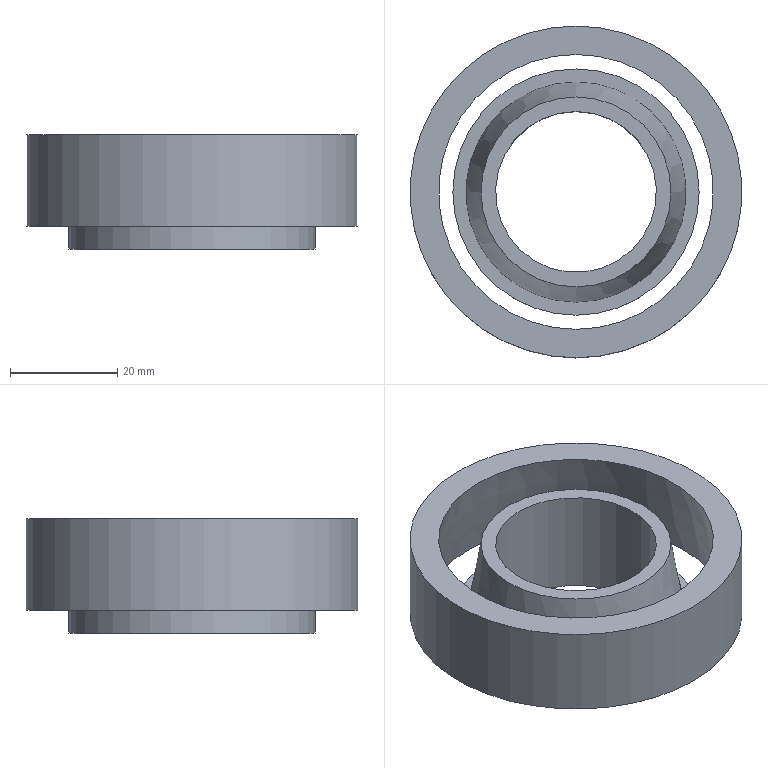Component | NX | GUNZIZGOUCHOU2 | 2 solids | 10 faces | box 61.88 x 61.88 x 21.26 mm | volume 22800 mm3 | plane 5 | cylinder 3 | cone 2 | commonest cylinder face diameters 61.88 x1 30 x1 45.92 x1
STEP:
#1=CARTESIAN_POINT('',(0.,0.,0.));
#2=DIRECTION('',(0.,0.,1.));
#3=DIRECTION('',(1.,0.,0.));
#4=AXIS2_PLACEMENT_3D('',#1,#2,#3);
#5=CARTESIAN_POINT('',(0.,28.646,365.26));
#6=VERTEX_POINT('',#5);
#7=CARTESIAN_POINT('',(0.,0.,365.26));
#8=DIRECTION('',(0.,0.,-1.));
#9=DIRECTION('',(0.,1.,0.));
#10=AXIS2_PLACEMENT_3D('',#7,#8,#9);
#11=CIRCLE('',#10,28.646);
#12=CARTESIAN_POINT('',(0.,0.,366.664));
#13=DIRECTION('',(0.,0.,-1.));
#14=DIRECTION('',(0.,1.,0.));
#15=AXIS2_PLACEMENT_3D('',#12,#13,#14);
#16=CONICAL_SURFACE('',#15,28.396,0.1764);
#17=CARTESIAN_POINT('',(0.,1.404));
#18=DIRECTION('',(1.,0.));
#19=VECTOR('',#18,1.);
#20=LINE('',#17,#19);
#21=(GEOMETRIC_REPRESENTATION_CONTEXT(2)PARAMETRIC_REPRESENTATION_CONTEXT()REPRESENTATION_CONTEXT('',''));
#22=DEFINITIONAL_REPRESENTATION('',(#20),#21);
#23=PCURVE('',#16,#22);
#24=CARTESIAN_POINT('',(28.646,0.,365.26));
#25=DIRECTION('',(0.,0.,-1.));
#26=DIRECTION('',(0.,1.,0.));
#27=AXIS2_PLACEMENT_3D('',#24,#25,#26);
#28=PLANE('',#27);
#29=CARTESIAN_POINT('',(0.,-28.646));
#30=DIRECTION('',(1.,0.));
#31=AXIS2_PLACEMENT_2D('',#29,#30);
#32=CIRCLE('',#31,28.646);
#33=(GEOMETRIC_REPRESENTATION_CONTEXT(2)PARAMETRIC_REPRESENTATION_CONTEXT()REPRESENTATION_CONTEXT('',''));
#34=DEFINITIONAL_REPRESENTATION('',(#32),#33);
#35=PCURVE('',#28,#34);
#36=SURFACE_CURVE('',#11,(#23,#35),.PCURVE_S1.);
#37=EDGE_CURVE('',#6,#6,#36,.T.);
#38=ORIENTED_EDGE('',*,*,#37,.F.);
#39=CARTESIAN_POINT('',(0.,25.616,382.26));
#40=VERTEX_POINT('',#39);
#41=CARTESIAN_POINT('',(-0.,25.616,382.26));
#42=CARTESIAN_POINT('',(-0.,28.646,365.26));
#43=B_SPLINE_CURVE_WITH_KNOTS('',1,(#41,#42),.UNSPECIFIED.,.F.,.F.,(2,2),(-15.842,1.426),.PIECEWISE_BEZIER_KNOTS.);
#44=CARTESIAN_POINT('',(0.,0.));
#45=DIRECTION('',(0.,1.));
#46=VECTOR('',#45,1.);
#47=LINE('',#44,#46);
#48=(GEOMETRIC_REPRESENTATION_CONTEXT(2)PARAMETRIC_REPRESENTATION_CONTEXT()REPRESENTATION_CONTEXT('',''));
#49=DEFINITIONAL_REPRESENTATION('',(#47),#48);
#50=PCURVE('',#16,#49);
#51=CARTESIAN_POINT('',(6.283,0.));
#52=DIRECTION('',(0.,1.));
#53=VECTOR('',#52,1.);
#54=LINE('',#51,#53);
#55=(GEOMETRIC_REPRESENTATION_CONTEXT(2)PARAMETRIC_REPRESENTATION_CONTEXT()REPRESENTATION_CONTEXT('',''));
#56=DEFINITIONAL_REPRESENTATION('',(#54),#55);
#57=PCURVE('',#16,#56);
#58=SEAM_CURVE('',#43,(#50,#57),.PCURVE_S1.);
#59=EDGE_CURVE('',#40,#6,#58,.T.);
#60=ORIENTED_EDGE('',*,*,#59,.F.);
#61=CARTESIAN_POINT('',(0.,0.,382.26));
#62=DIRECTION('',(0.,0.,-1.));
#63=DIRECTION('',(0.,1.,0.));
#64=AXIS2_PLACEMENT_3D('',#61,#62,#63);
#65=CIRCLE('',#64,25.616);
#66=CARTESIAN_POINT('',(0.,-15.596));
#67=DIRECTION('',(1.,0.));
#68=VECTOR('',#67,1.);
#69=LINE('',#66,#68);
#70=(GEOMETRIC_REPRESENTATION_CONTEXT(2)PARAMETRIC_REPRESENTATION_CONTEXT()REPRESENTATION_CONTEXT('',''));
#71=DEFINITIONAL_REPRESENTATION('',(#69),#70);
#72=PCURVE('',#16,#71);
#73=CARTESIAN_POINT('',(27.255,0.,382.26));
#74=DIRECTION('',(0.,0.,1.));
#75=DIRECTION('',(0.,-1.,0.));
#76=AXIS2_PLACEMENT_3D('',#73,#74,#75);
#77=PLANE('',#76);
#78=CARTESIAN_POINT('',(-25.616,-27.255));
#79=CARTESIAN_POINT('',(-25.616,17.113));
#80=CARTESIAN_POINT('',(12.808,-5.071));
#81=CARTESIAN_POINT('',(51.232,-27.255));
#82=CARTESIAN_POINT('',(12.808,-49.439));
#83=CARTESIAN_POINT('',(-25.616,-71.623));
#84=CARTESIAN_POINT('',(-25.616,-27.255));
#85=(BOUNDED_CURVE()B_SPLINE_CURVE(2,(#78,#79,#80,#81,#82,#83,#84),.UNSPECIFIED.,.T.,.F.)B_SPLINE_CURVE_WITH_KNOTS((1,2,2,2,2,1),(-2.094,0.,2.094,4.189,6.283,8.378),.UNSPECIFIED.)CURVE()GEOMETRIC_REPRESENTATION_ITEM()RATIONAL_B_SPLINE_CURVE((1.,0.5,1.,0.5,1.,0.5,1.))REPRESENTATION_ITEM(''));
#86=(GEOMETRIC_REPRESENTATION_CONTEXT(2)PARAMETRIC_REPRESENTATION_CONTEXT()REPRESENTATION_CONTEXT('',''));
#87=DEFINITIONAL_REPRESENTATION('',(#85),#86);
#88=PCURVE('',#77,#87);
#89=SURFACE_CURVE('',#65,(#72,#88),.PCURVE_S1.);
#90=EDGE_CURVE('',#40,#40,#89,.T.);
#91=ORIENTED_EDGE('',*,*,#90,.T.);
#92=ORIENTED_EDGE('',*,*,#59,.T.);
#93=EDGE_LOOP('',(#38,#60,#91,#92));
#94=FACE_BOUND('',#93,.F.);
#95=ADVANCED_FACE('',(#94),#16,.F.);
#96=CARTESIAN_POINT('',(0.,30.94,365.26));
#97=VERTEX_POINT('',#96);
#98=CARTESIAN_POINT('',(0.,0.,365.26));
#99=DIRECTION('',(0.,0.,-1.));
#100=DIRECTION('',(0.,1.,0.));
#101=AXIS2_PLACEMENT_3D('',#98,#99,#100);
#102=CIRCLE('',#101,30.94);
#103=CARTESIAN_POINT('',(0.,-28.646));
#104=DIRECTION('',(1.,0.));
#105=AXIS2_PLACEMENT_2D('',#103,#104);
#106=CIRCLE('',#105,30.94);
#107=(GEOMETRIC_REPRESENTATION_CONTEXT(2)PARAMETRIC_REPRESENTATION_CONTEXT()REPRESENTATION_CONTEXT('',''));
#108=DEFINITIONAL_REPRESENTATION('',(#106),#107);
#109=PCURVE('',#28,#108);
#110=CARTESIAN_POINT('',(0.,0.,361.));
#111=DIRECTION('',(0.,0.,-1.));
#112=DIRECTION('',(0.,1.,0.));
#113=AXIS2_PLACEMENT_3D('',#110,#111,#112);
#114=CYLINDRICAL_SURFACE('',#113,30.94);
#115=CARTESIAN_POINT('',(0.,-4.26));
#116=DIRECTION('',(1.,0.));
#117=VECTOR('',#116,1.);
#118=LINE('',#115,#117);
#119=(GEOMETRIC_REPRESENTATION_CONTEXT(2)PARAMETRIC_REPRESENTATION_CONTEXT()REPRESENTATION_CONTEXT('',''));
#120=DEFINITIONAL_REPRESENTATION('',(#118),#119);
#121=PCURVE('',#114,#120);
#122=SURFACE_CURVE('',#102,(#109,#121),.PCURVE_S1.);
#123=EDGE_CURVE('',#97,#97,#122,.T.);
#124=ORIENTED_EDGE('',*,*,#123,.T.);
#125=EDGE_LOOP('',(#124));
#126=FACE_BOUND('',#125,.T.);
#127=ORIENTED_EDGE('',*,*,#37,.F.);
#128=EDGE_LOOP('',(#127));
#129=FACE_BOUND('',#128,.T.);
#130=ADVANCED_FACE('',(#126,#129),#28,.T.);
#131=CARTESIAN_POINT('',(0.,30.94,382.26));
#132=VERTEX_POINT('',#131);
#133=CARTESIAN_POINT('',(0.,0.,382.26));
#134=DIRECTION('',(0.,0.,-1.));
#135=DIRECTION('',(0.,1.,0.));
#136=AXIS2_PLACEMENT_3D('',#133,#134,#135);
#137=CIRCLE('',#136,30.94);
#138=CARTESIAN_POINT('',(0.,-21.26));
#139=DIRECTION('',(1.,0.));
#140=VECTOR('',#139,1.);
#141=LINE('',#138,#140);
#142=(GEOMETRIC_REPRESENTATION_CONTEXT(2)PARAMETRIC_REPRESENTATION_CONTEXT()REPRESENTATION_CONTEXT('',''));
#143=DEFINITIONAL_REPRESENTATION('',(#141),#142);
#144=PCURVE('',#114,#143);
#145=CARTESIAN_POINT('',(-30.94,-27.255));
#146=CARTESIAN_POINT('',(-30.94,26.334));
#147=CARTESIAN_POINT('',(15.47,-0.4604));
#148=CARTESIAN_POINT('',(61.88,-27.255));
#149=CARTESIAN_POINT('',(15.47,-54.05));
#150=CARTESIAN_POINT('',(-30.94,-80.845));
#151=CARTESIAN_POINT('',(-30.94,-27.255));
#152=(BOUNDED_CURVE()B_SPLINE_CURVE(2,(#145,#146,#147,#148,#149,#150,#151),.UNSPECIFIED.,.T.,.F.)B_SPLINE_CURVE_WITH_KNOTS((1,2,2,2,2,1),(-2.094,0.,2.094,4.189,6.283,8.378),.UNSPECIFIED.)CURVE()GEOMETRIC_REPRESENTATION_ITEM()RATIONAL_B_SPLINE_CURVE((1.,0.5,1.,0.5,1.,0.5,1.))REPRESENTATION_ITEM(''));
#153=(GEOMETRIC_REPRESENTATION_CONTEXT(2)PARAMETRIC_REPRESENTATION_CONTEXT()REPRESENTATION_CONTEXT('',''));
#154=DEFINITIONAL_REPRESENTATION('',(#152),#153);
#155=PCURVE('',#77,#154);
#156=SURFACE_CURVE('',#137,(#144,#155),.PCURVE_S1.);
#157=EDGE_CURVE('',#132,#132,#156,.T.);
#158=ORIENTED_EDGE('',*,*,#157,.T.);
#159=CARTESIAN_POINT('',(0.,30.94,382.26));
#160=CARTESIAN_POINT('',(0.,30.94,365.26));
#161=B_SPLINE_CURVE_WITH_KNOTS('',1,(#159,#160),.UNSPECIFIED.,.F.,.F.,(2,2),(-21.26,-4.26),.PIECEWISE_BEZIER_KNOTS.);
#162=CARTESIAN_POINT('',(6.283,0.));
#163=DIRECTION('',(0.,1.));
#164=VECTOR('',#163,1.);
#165=LINE('',#162,#164);
#166=(GEOMETRIC_REPRESENTATION_CONTEXT(2)PARAMETRIC_REPRESENTATION_CONTEXT()REPRESENTATION_CONTEXT('',''));
#167=DEFINITIONAL_REPRESENTATION('',(#165),#166);
#168=PCURVE('',#114,#167);
#169=CARTESIAN_POINT('',(0.,0.));
#170=DIRECTION('',(0.,1.));
#171=VECTOR('',#170,1.);
#172=LINE('',#169,#171);
#173=(GEOMETRIC_REPRESENTATION_CONTEXT(2)PARAMETRIC_REPRESENTATION_CONTEXT()REPRESENTATION_CONTEXT('',''));
#174=DEFINITIONAL_REPRESENTATION('',(#172),#173);
#175=PCURVE('',#114,#174);
#176=SEAM_CURVE('',#161,(#168,#175),.PCURVE_S1.);
#177=EDGE_CURVE('',#132,#97,#176,.T.);
#178=ORIENTED_EDGE('',*,*,#177,.T.);
#179=ORIENTED_EDGE('',*,*,#123,.F.);
#180=ORIENTED_EDGE('',*,*,#177,.F.);
#181=EDGE_LOOP('',(#158,#178,#179,#180));
#182=FACE_BOUND('',#181,.T.);
#183=ADVANCED_FACE('',(#182),#114,.T.);
#184=ORIENTED_EDGE('',*,*,#90,.T.);
#185=EDGE_LOOP('',(#184));
#186=FACE_BOUND('',#185,.T.);
#187=ORIENTED_EDGE('',*,*,#157,.F.);
#188=EDGE_LOOP('',(#187));
#189=FACE_BOUND('',#188,.T.);
#190=ADVANCED_FACE('',(#186,#189),#77,.T.);
#191=CLOSED_SHELL('',(#95,#130,#183,#190));
#192=MANIFOLD_SOLID_BREP('',#191);
#193=(LENGTH_UNIT()NAMED_UNIT(*)SI_UNIT(.MILLI.,.METRE.));
#194=UNCERTAINTY_MEASURE_WITH_UNIT(LENGTH_MEASURE(0.00001),#193,'','');
#195=(NAMED_UNIT(*)PLANE_ANGLE_UNIT()SI_UNIT($,.RADIAN.));
#196=(NAMED_UNIT(*)SI_UNIT($,.STERADIAN.)SOLID_ANGLE_UNIT());
#197=(GEOMETRIC_REPRESENTATION_CONTEXT(3)GLOBAL_UNCERTAINTY_ASSIGNED_CONTEXT((#194))GLOBAL_UNIT_ASSIGNED_CONTEXT((#193,#195,#196))REPRESENTATION_CONTEXT('',''));
#198=ADVANCED_BREP_SHAPE_REPRESENTATION('',(#4,#192),#197);
#199=CARTESIAN_POINT('',(0.,0.,0.));
#200=DIRECTION('',(0.,0.,1.));
#201=DIRECTION('',(1.,0.,0.));
#202=AXIS2_PLACEMENT_3D('',#199,#200,#201);
#203=CARTESIAN_POINT('',(0.,0.,0.));
#204=DIRECTION('',(0.,0.,1.));
#205=DIRECTION('',(1.,0.,0.));
#206=AXIS2_PLACEMENT_3D('',#203,#204,#205);
#207=(LENGTH_UNIT()NAMED_UNIT(*)SI_UNIT(.MILLI.,.METRE.));
#208=UNCERTAINTY_MEASURE_WITH_UNIT(LENGTH_MEASURE(0.00001),#207,'','');
#209=(NAMED_UNIT(*)PLANE_ANGLE_UNIT()SI_UNIT($,.RADIAN.));
#210=(NAMED_UNIT(*)SI_UNIT($,.STERADIAN.)SOLID_ANGLE_UNIT());
#211=(GEOMETRIC_REPRESENTATION_CONTEXT(3)GLOBAL_UNCERTAINTY_ASSIGNED_CONTEXT((#208))GLOBAL_UNIT_ASSIGNED_CONTEXT((#207,#209,#210))REPRESENTATION_CONTEXT('',''));
#212=SHAPE_REPRESENTATION('',(#4,#202,#206),#211);
#213=ITEM_DEFINED_TRANSFORMATION('','',#4,#202);
#214=(REPRESENTATION_RELATIONSHIP('','',#198,#212)REPRESENTATION_RELATIONSHIP_WITH_TRANSFORMATION(#213)SHAPE_REPRESENTATION_RELATIONSHIP());
#215=CARTESIAN_POINT('',(0.,15.,381.02));
#216=VERTEX_POINT('',#215);
#217=CARTESIAN_POINT('',(0.,0.,381.02));
#218=DIRECTION('',(0.,0.,-1.));
#219=DIRECTION('',(0.,1.,0.));
#220=AXIS2_PLACEMENT_3D('',#217,#218,#219);
#221=CIRCLE('',#220,15.);
#222=CARTESIAN_POINT('',(17.711,0.,381.02));
#223=DIRECTION('',(0.,0.,1.));
#224=DIRECTION('',(0.,-1.,0.));
#225=AXIS2_PLACEMENT_3D('',#222,#223,#224);
#226=PLANE('',#225);
#227=CARTESIAN_POINT('',(-15.,-17.711));
#228=CARTESIAN_POINT('',(-15.,8.27));
#229=CARTESIAN_POINT('',(7.5,-4.72));
#230=CARTESIAN_POINT('',(30.,-17.711));
#231=CARTESIAN_POINT('',(7.5,-30.701));
#232=CARTESIAN_POINT('',(-15.,-43.691));
#233=CARTESIAN_POINT('',(-15.,-17.711));
#234=(BOUNDED_CURVE()B_SPLINE_CURVE(2,(#227,#228,#229,#230,#231,#232,#233),.UNSPECIFIED.,.T.,.F.)B_SPLINE_CURVE_WITH_KNOTS((1,2,2,2,2,1),(-2.094,0.,2.094,4.189,6.283,8.378),.UNSPECIFIED.)CURVE()GEOMETRIC_REPRESENTATION_ITEM()RATIONAL_B_SPLINE_CURVE((1.,0.5,1.,0.5,1.,0.5,1.))REPRESENTATION_ITEM(''));
#235=(GEOMETRIC_REPRESENTATION_CONTEXT(2)PARAMETRIC_REPRESENTATION_CONTEXT()REPRESENTATION_CONTEXT('',''));
#236=DEFINITIONAL_REPRESENTATION('',(#234),#235);
#237=PCURVE('',#226,#236);
#238=CARTESIAN_POINT('',(0.,0.,361.));
#239=DIRECTION('',(0.,0.,-1.));
#240=DIRECTION('',(0.,1.,0.));
#241=AXIS2_PLACEMENT_3D('',#238,#239,#240);
#242=CYLINDRICAL_SURFACE('',#241,15.);
#243=CARTESIAN_POINT('',(0.,-20.02));
#244=DIRECTION('',(1.,0.));
#245=VECTOR('',#244,1.);
#246=LINE('',#243,#245);
#247=(GEOMETRIC_REPRESENTATION_CONTEXT(2)PARAMETRIC_REPRESENTATION_CONTEXT()REPRESENTATION_CONTEXT('',''));
#248=DEFINITIONAL_REPRESENTATION('',(#246),#247);
#249=PCURVE('',#242,#248);
#250=SURFACE_CURVE('',#221,(#237,#249),.PCURVE_S1.);
#251=EDGE_CURVE('',#216,#216,#250,.T.);
#252=ORIENTED_EDGE('',*,*,#251,.T.);
#253=EDGE_LOOP('',(#252));
#254=FACE_BOUND('',#253,.T.);
#255=CARTESIAN_POINT('',(0.,17.711,381.02));
#256=VERTEX_POINT('',#255);
#257=CARTESIAN_POINT('',(0.,0.,381.02));
#258=DIRECTION('',(0.,0.,-1.));
#259=DIRECTION('',(0.,1.,0.));
#260=AXIS2_PLACEMENT_3D('',#257,#258,#259);
#261=CIRCLE('',#260,17.711);
#262=CARTESIAN_POINT('',(-17.711,-17.711));
#263=CARTESIAN_POINT('',(-17.711,12.965));
#264=CARTESIAN_POINT('',(8.855,-2.373));
#265=CARTESIAN_POINT('',(35.421,-17.711));
#266=CARTESIAN_POINT('',(8.855,-33.049));
#267=CARTESIAN_POINT('',(-17.711,-48.387));
#268=CARTESIAN_POINT('',(-17.711,-17.711));
#269=(BOUNDED_CURVE()B_SPLINE_CURVE(2,(#262,#263,#264,#265,#266,#267,#268),.UNSPECIFIED.,.T.,.F.)B_SPLINE_CURVE_WITH_KNOTS((1,2,2,2,2,1),(-2.094,0.,2.094,4.189,6.283,8.378),.UNSPECIFIED.)CURVE()GEOMETRIC_REPRESENTATION_ITEM()RATIONAL_B_SPLINE_CURVE((1.,0.5,1.,0.5,1.,0.5,1.))REPRESENTATION_ITEM(''));
#270=(GEOMETRIC_REPRESENTATION_CONTEXT(2)PARAMETRIC_REPRESENTATION_CONTEXT()REPRESENTATION_CONTEXT('',''));
#271=DEFINITIONAL_REPRESENTATION('',(#269),#270);
#272=PCURVE('',#226,#271);
#273=CARTESIAN_POINT('',(0.,0.,365.26));
#274=DIRECTION('',(0.,0.,-1.));
#275=DIRECTION('',(0.,1.,0.));
#276=AXIS2_PLACEMENT_3D('',#273,#274,#275);
#277=CONICAL_SURFACE('',#276,20.52,0.1764);
#278=CARTESIAN_POINT('',(0.,-15.76));
#279=DIRECTION('',(1.,0.));
#280=VECTOR('',#279,1.);
#281=LINE('',#278,#280);
#282=(GEOMETRIC_REPRESENTATION_CONTEXT(2)PARAMETRIC_REPRESENTATION_CONTEXT()REPRESENTATION_CONTEXT('',''));
#283=DEFINITIONAL_REPRESENTATION('',(#281),#282);
#284=PCURVE('',#277,#283);
#285=SURFACE_CURVE('',#261,(#272,#284),.PCURVE_S1.);
#286=EDGE_CURVE('',#256,#256,#285,.T.);
#287=ORIENTED_EDGE('',*,*,#286,.F.);
#288=EDGE_LOOP('',(#287));
#289=FACE_BOUND('',#288,.T.);
#290=ADVANCED_FACE('',(#254,#289),#226,.T.);
#291=CARTESIAN_POINT('',(0.,15.,361.));
#292=VERTEX_POINT('',#291);
#293=CARTESIAN_POINT('',(0.,0.,361.));
#294=DIRECTION('',(0.,0.,-1.));
#295=DIRECTION('',(0.,1.,0.));
#296=AXIS2_PLACEMENT_3D('',#293,#294,#295);
#297=CIRCLE('',#296,15.);
#298=CARTESIAN_POINT('',(0.,0.));
#299=DIRECTION('',(1.,0.));
#300=VECTOR('',#299,1.);
#301=LINE('',#298,#300);
#302=(GEOMETRIC_REPRESENTATION_CONTEXT(2)PARAMETRIC_REPRESENTATION_CONTEXT()REPRESENTATION_CONTEXT('',''));
#303=DEFINITIONAL_REPRESENTATION('',(#301),#302);
#304=PCURVE('',#242,#303);
#305=CARTESIAN_POINT('',(15.,0.,361.));
#306=DIRECTION('',(0.,0.,-1.));
#307=DIRECTION('',(0.,1.,0.));
#308=AXIS2_PLACEMENT_3D('',#305,#306,#307);
#309=PLANE('',#308);
#310=CARTESIAN_POINT('',(0.,-15.));
#311=DIRECTION('',(1.,0.));
#312=AXIS2_PLACEMENT_2D('',#310,#311);
#313=CIRCLE('',#312,15.);
#314=(GEOMETRIC_REPRESENTATION_CONTEXT(2)PARAMETRIC_REPRESENTATION_CONTEXT()REPRESENTATION_CONTEXT('',''));
#315=DEFINITIONAL_REPRESENTATION('',(#313),#314);
#316=PCURVE('',#309,#315);
#317=SURFACE_CURVE('',#297,(#304,#316),.PCURVE_S1.);
#318=EDGE_CURVE('',#292,#292,#317,.T.);
#319=ORIENTED_EDGE('',*,*,#318,.F.);
#320=CARTESIAN_POINT('',(-0.,15.,381.02));
#321=CARTESIAN_POINT('',(-0.,15.,361.));
#322=B_SPLINE_CURVE_WITH_KNOTS('',1,(#320,#321),.UNSPECIFIED.,.F.,.F.,(2,2),(-20.02,0.),.PIECEWISE_BEZIER_KNOTS.);
#323=CARTESIAN_POINT('',(0.,0.));
#324=DIRECTION('',(0.,1.));
#325=VECTOR('',#324,1.);
#326=LINE('',#323,#325);
#327=(GEOMETRIC_REPRESENTATION_CONTEXT(2)PARAMETRIC_REPRESENTATION_CONTEXT()REPRESENTATION_CONTEXT('',''));
#328=DEFINITIONAL_REPRESENTATION('',(#326),#327);
#329=PCURVE('',#242,#328);
#330=CARTESIAN_POINT('',(6.283,0.));
#331=DIRECTION('',(0.,1.));
#332=VECTOR('',#331,1.);
#333=LINE('',#330,#332);
#334=(GEOMETRIC_REPRESENTATION_CONTEXT(2)PARAMETRIC_REPRESENTATION_CONTEXT()REPRESENTATION_CONTEXT('',''));
#335=DEFINITIONAL_REPRESENTATION('',(#333),#334);
#336=PCURVE('',#242,#335);
#337=SEAM_CURVE('',#322,(#329,#336),.PCURVE_S1.);
#338=EDGE_CURVE('',#216,#292,#337,.T.);
#339=ORIENTED_EDGE('',*,*,#338,.F.);
#340=ORIENTED_EDGE('',*,*,#251,.T.);
#341=ORIENTED_EDGE('',*,*,#338,.T.);
#342=EDGE_LOOP('',(#319,#339,#340,#341));
#343=FACE_BOUND('',#342,.F.);
#344=ADVANCED_FACE('',(#343),#242,.F.);
#345=CARTESIAN_POINT('',(0.,22.96,361.));
#346=VERTEX_POINT('',#345);
#347=CARTESIAN_POINT('',(0.,0.,361.));
#348=DIRECTION('',(0.,0.,-1.));
#349=DIRECTION('',(0.,1.,0.));
#350=AXIS2_PLACEMENT_3D('',#347,#348,#349);
#351=CIRCLE('',#350,22.96);
#352=CARTESIAN_POINT('',(0.,-15.));
#353=DIRECTION('',(1.,0.));
#354=AXIS2_PLACEMENT_2D('',#352,#353);
#355=CIRCLE('',#354,22.96);
#356=(GEOMETRIC_REPRESENTATION_CONTEXT(2)PARAMETRIC_REPRESENTATION_CONTEXT()REPRESENTATION_CONTEXT('',''));
#357=DEFINITIONAL_REPRESENTATION('',(#355),#356);
#358=PCURVE('',#309,#357);
#359=CARTESIAN_POINT('',(0.,0.,361.));
#360=DIRECTION('',(0.,0.,-1.));
#361=DIRECTION('',(0.,1.,0.));
#362=AXIS2_PLACEMENT_3D('',#359,#360,#361);
#363=CYLINDRICAL_SURFACE('',#362,22.96);
#364=CARTESIAN_POINT('',(0.,0.));
#365=DIRECTION('',(1.,0.));
#366=VECTOR('',#365,1.);
#367=LINE('',#364,#366);
#368=(GEOMETRIC_REPRESENTATION_CONTEXT(2)PARAMETRIC_REPRESENTATION_CONTEXT()REPRESENTATION_CONTEXT('',''));
#369=DEFINITIONAL_REPRESENTATION('',(#367),#368);
#370=PCURVE('',#363,#369);
#371=SURFACE_CURVE('',#351,(#358,#370),.PCURVE_S1.);
#372=EDGE_CURVE('',#346,#346,#371,.T.);
#373=ORIENTED_EDGE('',*,*,#372,.T.);
#374=EDGE_LOOP('',(#373));
#375=FACE_BOUND('',#374,.T.);
#376=ORIENTED_EDGE('',*,*,#318,.F.);
#377=EDGE_LOOP('',(#376));
#378=FACE_BOUND('',#377,.T.);
#379=ADVANCED_FACE('',(#375,#378),#309,.T.);
#380=CARTESIAN_POINT('',(0.,22.96,365.26));
#381=VERTEX_POINT('',#380);
#382=CARTESIAN_POINT('',(0.,0.,365.26));
#383=DIRECTION('',(0.,0.,-1.));
#384=DIRECTION('',(0.,1.,0.));
#385=AXIS2_PLACEMENT_3D('',#382,#383,#384);
#386=CIRCLE('',#385,22.96);
#387=CARTESIAN_POINT('',(0.,-4.26));
#388=DIRECTION('',(1.,0.));
#389=VECTOR('',#388,1.);
#390=LINE('',#387,#389);
#391=(GEOMETRIC_REPRESENTATION_CONTEXT(2)PARAMETRIC_REPRESENTATION_CONTEXT()REPRESENTATION_CONTEXT('',''));
#392=DEFINITIONAL_REPRESENTATION('',(#390),#391);
#393=PCURVE('',#363,#392);
#394=CARTESIAN_POINT('',(22.96,0.,365.26));
#395=DIRECTION('',(0.,0.,1.));
#396=DIRECTION('',(0.,-1.,0.));
#397=AXIS2_PLACEMENT_3D('',#394,#395,#396);
#398=PLANE('',#397);
#399=CARTESIAN_POINT('',(-22.96,-22.96));
#400=CARTESIAN_POINT('',(-22.96,16.808));
#401=CARTESIAN_POINT('',(11.48,-3.076));
#402=CARTESIAN_POINT('',(45.92,-22.96));
#403=CARTESIAN_POINT('',(11.48,-42.844));
#404=CARTESIAN_POINT('',(-22.96,-62.728));
#405=CARTESIAN_POINT('',(-22.96,-22.96));
#406=(BOUNDED_CURVE()B_SPLINE_CURVE(2,(#399,#400,#401,#402,#403,#404,#405),.UNSPECIFIED.,.T.,.F.)B_SPLINE_CURVE_WITH_KNOTS((1,2,2,2,2,1),(-2.094,0.,2.094,4.189,6.283,8.378),.UNSPECIFIED.)CURVE()GEOMETRIC_REPRESENTATION_ITEM()RATIONAL_B_SPLINE_CURVE((1.,0.5,1.,0.5,1.,0.5,1.))REPRESENTATION_ITEM(''));
#407=(GEOMETRIC_REPRESENTATION_CONTEXT(2)PARAMETRIC_REPRESENTATION_CONTEXT()REPRESENTATION_CONTEXT('',''));
#408=DEFINITIONAL_REPRESENTATION('',(#406),#407);
#409=PCURVE('',#398,#408);
#410=SURFACE_CURVE('',#386,(#393,#409),.PCURVE_S1.);
#411=EDGE_CURVE('',#381,#381,#410,.T.);
#412=ORIENTED_EDGE('',*,*,#411,.T.);
#413=CARTESIAN_POINT('',(0.,22.96,365.26));
#414=CARTESIAN_POINT('',(0.,22.96,361.));
#415=B_SPLINE_CURVE_WITH_KNOTS('',1,(#413,#414),.UNSPECIFIED.,.F.,.F.,(2,2),(-4.26,0.),.PIECEWISE_BEZIER_KNOTS.);
#416=CARTESIAN_POINT('',(6.283,0.));
#417=DIRECTION('',(0.,1.));
#418=VECTOR('',#417,1.);
#419=LINE('',#416,#418);
#420=(GEOMETRIC_REPRESENTATION_CONTEXT(2)PARAMETRIC_REPRESENTATION_CONTEXT()REPRESENTATION_CONTEXT('',''));
#421=DEFINITIONAL_REPRESENTATION('',(#419),#420);
#422=PCURVE('',#363,#421);
#423=CARTESIAN_POINT('',(0.,0.));
#424=DIRECTION('',(0.,1.));
#425=VECTOR('',#424,1.);
#426=LINE('',#423,#425);
#427=(GEOMETRIC_REPRESENTATION_CONTEXT(2)PARAMETRIC_REPRESENTATION_CONTEXT()REPRESENTATION_CONTEXT('',''));
#428=DEFINITIONAL_REPRESENTATION('',(#426),#427);
#429=PCURVE('',#363,#428);
#430=SEAM_CURVE('',#415,(#422,#429),.PCURVE_S1.);
#431=EDGE_CURVE('',#381,#346,#430,.T.);
#432=ORIENTED_EDGE('',*,*,#431,.T.);
#433=ORIENTED_EDGE('',*,*,#372,.F.);
#434=ORIENTED_EDGE('',*,*,#431,.F.);
#435=EDGE_LOOP('',(#412,#432,#433,#434));
#436=FACE_BOUND('',#435,.T.);
#437=ADVANCED_FACE('',(#436),#363,.T.);
#438=CARTESIAN_POINT('',(0.,20.52,365.26));
#439=VERTEX_POINT('',#438);
#440=CARTESIAN_POINT('',(0.,0.,365.26));
#441=DIRECTION('',(0.,0.,-1.));
#442=DIRECTION('',(0.,1.,0.));
#443=AXIS2_PLACEMENT_3D('',#440,#441,#442);
#444=CIRCLE('',#443,20.52);
#445=CARTESIAN_POINT('',(-20.52,-22.96));
#446=CARTESIAN_POINT('',(-20.52,12.582));
#447=CARTESIAN_POINT('',(10.26,-5.189));
#448=CARTESIAN_POINT('',(41.04,-22.96));
#449=CARTESIAN_POINT('',(10.26,-40.731));
#450=CARTESIAN_POINT('',(-20.52,-58.502));
#451=CARTESIAN_POINT('',(-20.52,-22.96));
#452=(BOUNDED_CURVE()B_SPLINE_CURVE(2,(#445,#446,#447,#448,#449,#450,#451),.UNSPECIFIED.,.T.,.F.)B_SPLINE_CURVE_WITH_KNOTS((1,2,2,2,2,1),(-2.094,0.,2.094,4.189,6.283,8.378),.UNSPECIFIED.)CURVE()GEOMETRIC_REPRESENTATION_ITEM()RATIONAL_B_SPLINE_CURVE((1.,0.5,1.,0.5,1.,0.5,1.))REPRESENTATION_ITEM(''));
#453=(GEOMETRIC_REPRESENTATION_CONTEXT(2)PARAMETRIC_REPRESENTATION_CONTEXT()REPRESENTATION_CONTEXT('',''));
#454=DEFINITIONAL_REPRESENTATION('',(#452),#453);
#455=PCURVE('',#398,#454);
#456=CARTESIAN_POINT('',(0.,0.));
#457=DIRECTION('',(1.,0.));
#458=VECTOR('',#457,1.);
#459=LINE('',#456,#458);
#460=(GEOMETRIC_REPRESENTATION_CONTEXT(2)PARAMETRIC_REPRESENTATION_CONTEXT()REPRESENTATION_CONTEXT('',''));
#461=DEFINITIONAL_REPRESENTATION('',(#459),#460);
#462=PCURVE('',#277,#461);
#463=SURFACE_CURVE('',#444,(#455,#462),.PCURVE_S1.);
#464=EDGE_CURVE('',#439,#439,#463,.T.);
#465=ORIENTED_EDGE('',*,*,#464,.T.);
#466=EDGE_LOOP('',(#465));
#467=FACE_BOUND('',#466,.T.);
#468=ORIENTED_EDGE('',*,*,#411,.F.);
#469=EDGE_LOOP('',(#468));
#470=FACE_BOUND('',#469,.T.);
#471=ADVANCED_FACE('',(#467,#470),#398,.T.);
#472=ORIENTED_EDGE('',*,*,#286,.T.);
#473=CARTESIAN_POINT('',(0.,17.711,381.02));
#474=CARTESIAN_POINT('',(0.,20.52,365.26));
#475=B_SPLINE_CURVE_WITH_KNOTS('',1,(#473,#474),.UNSPECIFIED.,.F.,.F.,(2,2),(-16.008,0.),.PIECEWISE_BEZIER_KNOTS.);
#476=CARTESIAN_POINT('',(6.283,0.));
#477=DIRECTION('',(0.,1.));
#478=VECTOR('',#477,1.);
#479=LINE('',#476,#478);
#480=(GEOMETRIC_REPRESENTATION_CONTEXT(2)PARAMETRIC_REPRESENTATION_CONTEXT()REPRESENTATION_CONTEXT('',''));
#481=DEFINITIONAL_REPRESENTATION('',(#479),#480);
#482=PCURVE('',#277,#481);
#483=CARTESIAN_POINT('',(0.,0.));
#484=DIRECTION('',(0.,1.));
#485=VECTOR('',#484,1.);
#486=LINE('',#483,#485);
#487=(GEOMETRIC_REPRESENTATION_CONTEXT(2)PARAMETRIC_REPRESENTATION_CONTEXT()REPRESENTATION_CONTEXT('',''));
#488=DEFINITIONAL_REPRESENTATION('',(#486),#487);
#489=PCURVE('',#277,#488);
#490=SEAM_CURVE('',#475,(#482,#489),.PCURVE_S1.);
#491=EDGE_CURVE('',#256,#439,#490,.T.);
#492=ORIENTED_EDGE('',*,*,#491,.T.);
#493=ORIENTED_EDGE('',*,*,#464,.F.);
#494=ORIENTED_EDGE('',*,*,#491,.F.);
#495=EDGE_LOOP('',(#472,#492,#493,#494));
#496=FACE_BOUND('',#495,.T.);
#497=ADVANCED_FACE('',(#496),#277,.T.);
#498=CLOSED_SHELL('',(#290,#344,#379,#437,#471,#497));
#499=MANIFOLD_SOLID_BREP('',#498);
#500=(LENGTH_UNIT()NAMED_UNIT(*)SI_UNIT(.MILLI.,.METRE.));
#501=UNCERTAINTY_MEASURE_WITH_UNIT(LENGTH_MEASURE(0.00001),#500,'','');
#502=(NAMED_UNIT(*)PLANE_ANGLE_UNIT()SI_UNIT($,.RADIAN.));
#503=(NAMED_UNIT(*)SI_UNIT($,.STERADIAN.)SOLID_ANGLE_UNIT());
#504=(GEOMETRIC_REPRESENTATION_CONTEXT(3)GLOBAL_UNCERTAINTY_ASSIGNED_CONTEXT((#501))GLOBAL_UNIT_ASSIGNED_CONTEXT((#500,#502,#503))REPRESENTATION_CONTEXT('',''));
#505=ADVANCED_BREP_SHAPE_REPRESENTATION('',(#4,#499),#504);
#506=ITEM_DEFINED_TRANSFORMATION('','',#4,#206);
#507=(REPRESENTATION_RELATIONSHIP('','',#505,#212)REPRESENTATION_RELATIONSHIP_WITH_TRANSFORMATION(#506)SHAPE_REPRESENTATION_RELATIONSHIP());